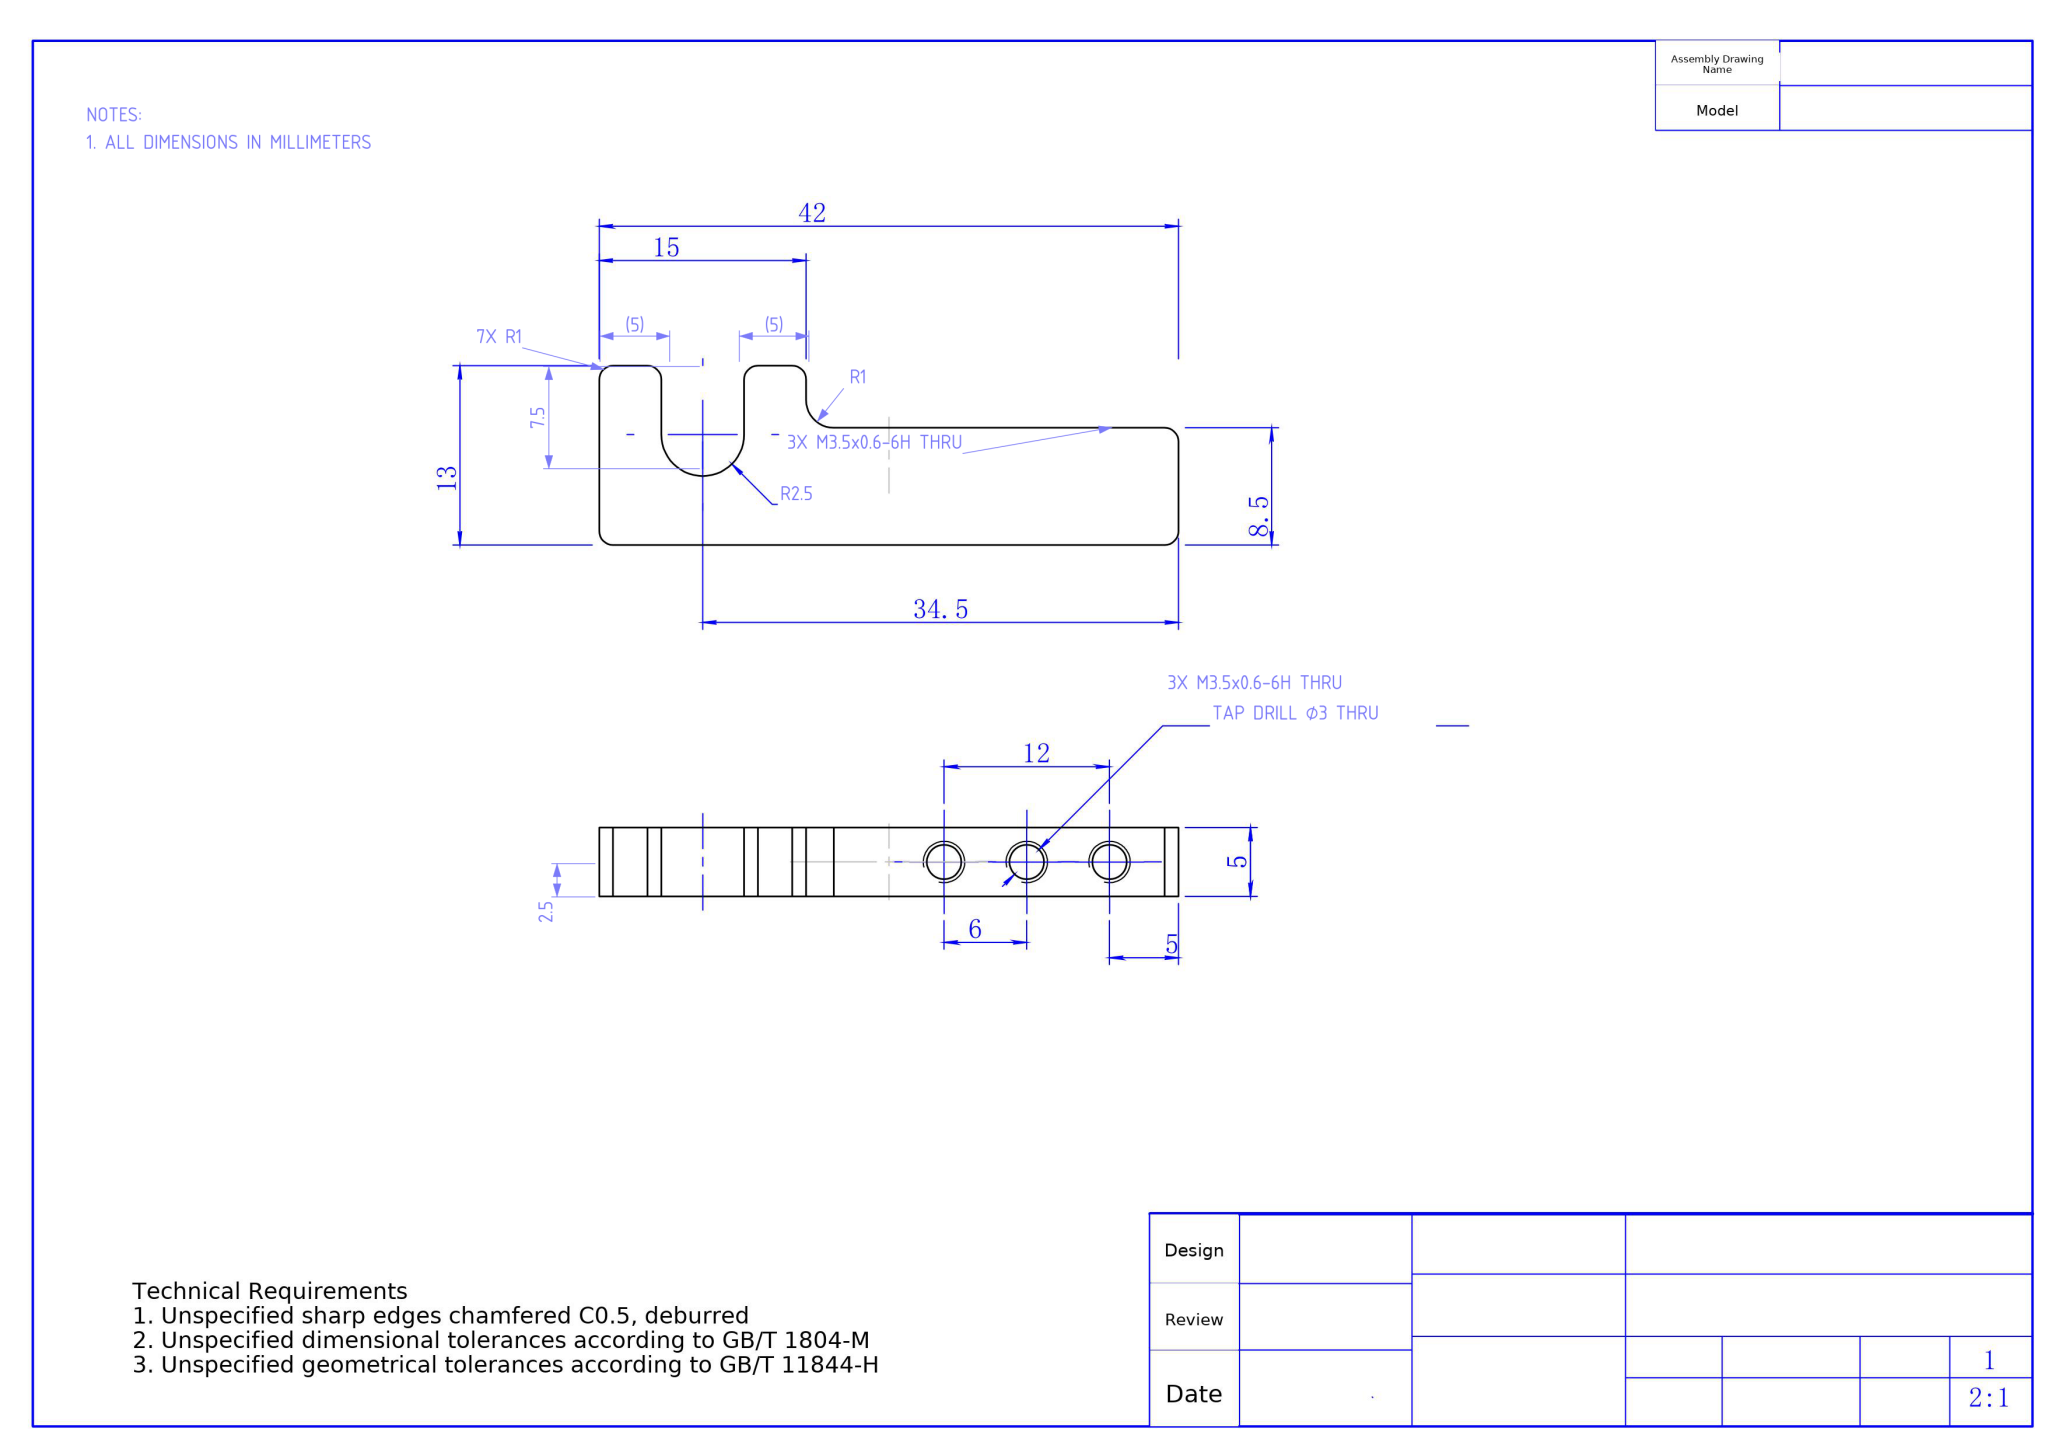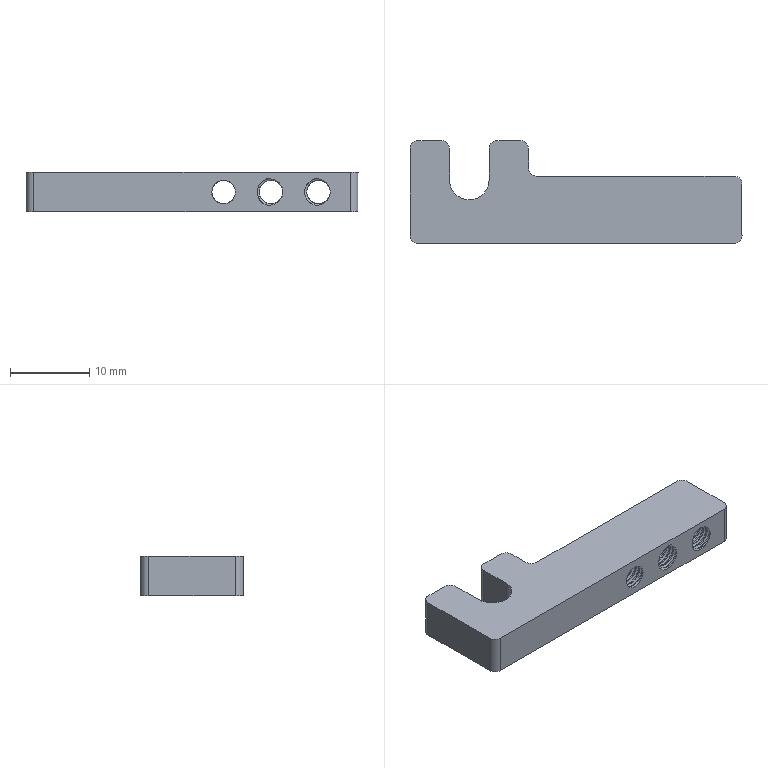Part | NX | mm | 1 solid | 35 faces | box 42 x 13.01 x 5.01 mm | volume 1854 mm3 | cylinder 15 | plane 14 | spline 6 | commonest cylinder face diameters 2 x8 3 x3 3.5 x3 5 x1